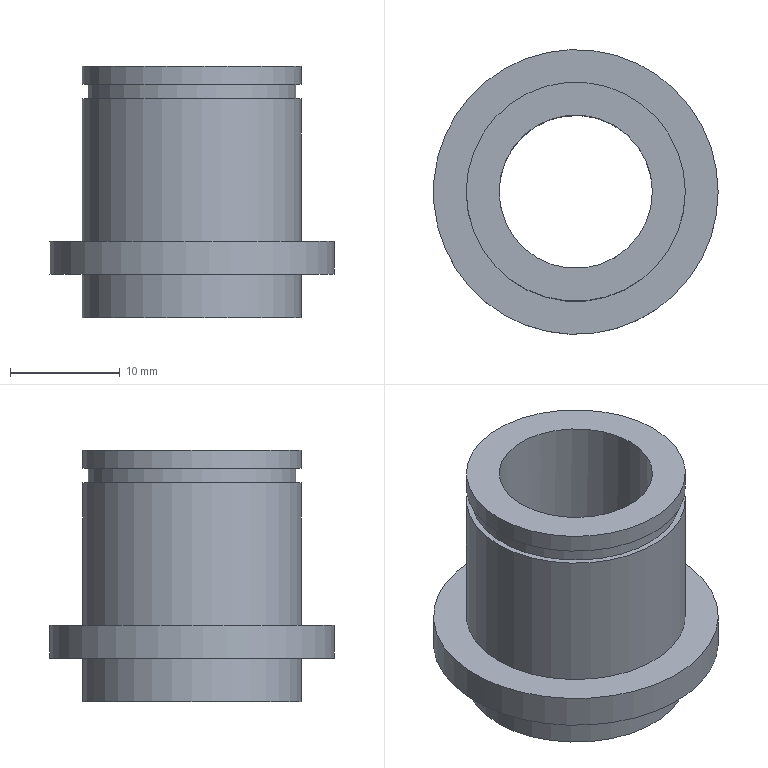Component | NX | 7 | 1 solid | 12 faces | box 26 x 26 x 23 mm | volume 4294 mm3 | plane 6 | cylinder 6 | commonest cylinder face diameters 20 x3 19 x1 26 x1 14 x1
STEP:
#1=CARTESIAN_POINT('',(0.,0.,0.));
#2=DIRECTION('',(0.,0.,1.));
#3=DIRECTION('',(1.,0.,0.));
#4=AXIS2_PLACEMENT_3D('',#1,#2,#3);
#5=CARTESIAN_POINT('',(-11.58,12.798,-36.));
#6=VERTEX_POINT('',#5);
#7=CARTESIAN_POINT('',(2.42,12.798,-36.));
#8=VERTEX_POINT('',#7);
#9=CARTESIAN_POINT('',(-4.58,12.798,-36.));
#10=DIRECTION('',(0.,0.,-1.));
#11=DIRECTION('',(-1.,0.,0.));
#12=AXIS2_PLACEMENT_3D('',#9,#10,#11);
#13=CIRCLE('',#12,7.);
#14=CARTESIAN_POINT('',(-4.58,2.798,-36.));
#15=DIRECTION('',(0.,0.,1.));
#16=DIRECTION('',(-1.,0.,0.));
#17=AXIS2_PLACEMENT_3D('',#14,#15,#16);
#18=PLANE('',#17);
#19=CARTESIAN_POINT('',(7.,-10.));
#20=CARTESIAN_POINT('',(7.,-22.124));
#21=CARTESIAN_POINT('',(-3.5,-16.062));
#22=CARTESIAN_POINT('',(-14.,-10.));
#23=CARTESIAN_POINT('',(-3.5,-3.938));
#24=CARTESIAN_POINT('',(7.,2.124));
#25=CARTESIAN_POINT('',(7.,-10.));
#26=(BOUNDED_CURVE()B_SPLINE_CURVE(2,(#19,#20,#21,#22,#23,#24,#25),.UNSPECIFIED.,.T.,.F.)B_SPLINE_CURVE_WITH_KNOTS((1,2,2,2,2,1),(-2.094,0.,2.094,4.189,6.283,8.378),.UNSPECIFIED.)CURVE()GEOMETRIC_REPRESENTATION_ITEM()RATIONAL_B_SPLINE_CURVE((1.,0.5,1.,0.5,1.,0.5,1.))REPRESENTATION_ITEM(''));
#27=(GEOMETRIC_REPRESENTATION_CONTEXT(2)PARAMETRIC_REPRESENTATION_CONTEXT()REPRESENTATION_CONTEXT('',''));
#28=DEFINITIONAL_REPRESENTATION('',(#26),#27);
#29=PCURVE('',#18,#28);
#30=CARTESIAN_POINT('',(-4.58,12.798,-23.5));
#31=DIRECTION('',(0.,0.,-1.));
#32=DIRECTION('',(1.,0.,0.));
#33=AXIS2_PLACEMENT_3D('',#30,#31,#32);
#34=CYLINDRICAL_SURFACE('',#33,7.);
#35=CARTESIAN_POINT('',(3.142,12.5));
#36=DIRECTION('',(1.,0.));
#37=VECTOR('',#36,1.);
#38=LINE('',#35,#37);
#39=(GEOMETRIC_REPRESENTATION_CONTEXT(2)PARAMETRIC_REPRESENTATION_CONTEXT()REPRESENTATION_CONTEXT('',''));
#40=DEFINITIONAL_REPRESENTATION('',(#38),#39);
#41=PCURVE('',#34,#40);
#42=SURFACE_CURVE('',#13,(#29,#41),.PCURVE_S1.);
#43=EDGE_CURVE('',#6,#8,#42,.T.);
#44=ORIENTED_EDGE('',*,*,#43,.T.);
#45=CARTESIAN_POINT('',(-4.58,12.798,-36.));
#46=DIRECTION('',(0.,0.,-1.));
#47=DIRECTION('',(-1.,0.,0.));
#48=AXIS2_PLACEMENT_3D('',#45,#46,#47);
#49=CIRCLE('',#48,7.);
#50=CARTESIAN_POINT('',(7.,-10.));
#51=CARTESIAN_POINT('',(7.,-22.124));
#52=CARTESIAN_POINT('',(-3.5,-16.062));
#53=CARTESIAN_POINT('',(-14.,-10.));
#54=CARTESIAN_POINT('',(-3.5,-3.938));
#55=CARTESIAN_POINT('',(7.,2.124));
#56=CARTESIAN_POINT('',(7.,-10.));
#57=(BOUNDED_CURVE()B_SPLINE_CURVE(2,(#50,#51,#52,#53,#54,#55,#56),.UNSPECIFIED.,.T.,.F.)B_SPLINE_CURVE_WITH_KNOTS((1,2,2,2,2,1),(-2.094,0.,2.094,4.189,6.283,8.378),.UNSPECIFIED.)CURVE()GEOMETRIC_REPRESENTATION_ITEM()RATIONAL_B_SPLINE_CURVE((1.,0.5,1.,0.5,1.,0.5,1.))REPRESENTATION_ITEM(''));
#58=(GEOMETRIC_REPRESENTATION_CONTEXT(2)PARAMETRIC_REPRESENTATION_CONTEXT()REPRESENTATION_CONTEXT('',''));
#59=DEFINITIONAL_REPRESENTATION('',(#57),#58);
#60=PCURVE('',#18,#59);
#61=CARTESIAN_POINT('',(-3.142,12.5));
#62=DIRECTION('',(1.,0.));
#63=VECTOR('',#62,1.);
#64=LINE('',#61,#63);
#65=(GEOMETRIC_REPRESENTATION_CONTEXT(2)PARAMETRIC_REPRESENTATION_CONTEXT()REPRESENTATION_CONTEXT('',''));
#66=DEFINITIONAL_REPRESENTATION('',(#64),#65);
#67=PCURVE('',#34,#66);
#68=SURFACE_CURVE('',#49,(#60,#67),.PCURVE_S1.);
#69=EDGE_CURVE('',#8,#6,#68,.T.);
#70=ORIENTED_EDGE('',*,*,#69,.T.);
#71=EDGE_LOOP('',(#44,#70));
#72=FACE_BOUND('',#71,.T.);
#73=CARTESIAN_POINT('',(5.42,12.798,-36.));
#74=VERTEX_POINT('',#73);
#75=CARTESIAN_POINT('',(-4.58,12.798,-36.));
#76=DIRECTION('',(0.,0.,-1.));
#77=DIRECTION('',(1.,0.,0.));
#78=AXIS2_PLACEMENT_3D('',#75,#76,#77);
#79=CIRCLE('',#78,10.);
#80=CARTESIAN_POINT('',(-10.,-10.));
#81=CARTESIAN_POINT('',(-10.,7.321));
#82=CARTESIAN_POINT('',(5.,-1.34));
#83=CARTESIAN_POINT('',(20.,-10.));
#84=CARTESIAN_POINT('',(5.,-18.66));
#85=CARTESIAN_POINT('',(-10.,-27.321));
#86=CARTESIAN_POINT('',(-10.,-10.));
#87=(BOUNDED_CURVE()B_SPLINE_CURVE(2,(#80,#81,#82,#83,#84,#85,#86),.UNSPECIFIED.,.T.,.F.)B_SPLINE_CURVE_WITH_KNOTS((1,2,2,2,2,1),(-2.094,0.,2.094,4.189,6.283,8.378),.UNSPECIFIED.)CURVE()GEOMETRIC_REPRESENTATION_ITEM()RATIONAL_B_SPLINE_CURVE((1.,0.5,1.,0.5,1.,0.5,1.))REPRESENTATION_ITEM(''));
#88=(GEOMETRIC_REPRESENTATION_CONTEXT(2)PARAMETRIC_REPRESENTATION_CONTEXT()REPRESENTATION_CONTEXT('',''));
#89=DEFINITIONAL_REPRESENTATION('',(#87),#88);
#90=PCURVE('',#18,#89);
#91=CARTESIAN_POINT('',(-4.58,12.798,-36.));
#92=DIRECTION('',(0.,0.,-1.));
#93=DIRECTION('',(1.,0.,0.));
#94=AXIS2_PLACEMENT_3D('',#91,#92,#93);
#95=CYLINDRICAL_SURFACE('',#94,10.);
#96=CARTESIAN_POINT('',(0.,0.));
#97=DIRECTION('',(1.,0.));
#98=VECTOR('',#97,1.);
#99=LINE('',#96,#98);
#100=(GEOMETRIC_REPRESENTATION_CONTEXT(2)PARAMETRIC_REPRESENTATION_CONTEXT()REPRESENTATION_CONTEXT('',''));
#101=DEFINITIONAL_REPRESENTATION('',(#99),#100);
#102=PCURVE('',#95,#101);
#103=SURFACE_CURVE('',#79,(#90,#102),.PCURVE_S1.);
#104=EDGE_CURVE('',#74,#74,#103,.T.);
#105=ORIENTED_EDGE('',*,*,#104,.F.);
#106=EDGE_LOOP('',(#105));
#107=FACE_BOUND('',#106,.T.);
#108=ADVANCED_FACE('',(#72,#107),#18,.T.);
#109=ORIENTED_EDGE('',*,*,#104,.T.);
#110=CARTESIAN_POINT('',(5.42,12.798,-37.65));
#111=VERTEX_POINT('',#110);
#112=CARTESIAN_POINT('',(5.42,12.798,-36.));
#113=CARTESIAN_POINT('',(5.42,12.798,-37.65));
#114=B_SPLINE_CURVE_WITH_KNOTS('',1,(#112,#113),.UNSPECIFIED.,.F.,.F.,(2,2),(0.,1.65),.PIECEWISE_BEZIER_KNOTS.);
#115=CARTESIAN_POINT('',(6.283,0.));
#116=DIRECTION('',(0.,1.));
#117=VECTOR('',#116,1.);
#118=LINE('',#115,#117);
#119=(GEOMETRIC_REPRESENTATION_CONTEXT(2)PARAMETRIC_REPRESENTATION_CONTEXT()REPRESENTATION_CONTEXT('',''));
#120=DEFINITIONAL_REPRESENTATION('',(#118),#119);
#121=PCURVE('',#95,#120);
#122=CARTESIAN_POINT('',(0.,0.));
#123=DIRECTION('',(0.,1.));
#124=VECTOR('',#123,1.);
#125=LINE('',#122,#124);
#126=(GEOMETRIC_REPRESENTATION_CONTEXT(2)PARAMETRIC_REPRESENTATION_CONTEXT()REPRESENTATION_CONTEXT('',''));
#127=DEFINITIONAL_REPRESENTATION('',(#125),#126);
#128=PCURVE('',#95,#127);
#129=SEAM_CURVE('',#114,(#121,#128),.PCURVE_S1.);
#130=EDGE_CURVE('',#74,#111,#129,.T.);
#131=ORIENTED_EDGE('',*,*,#130,.T.);
#132=CARTESIAN_POINT('',(-4.58,12.798,-37.65));
#133=DIRECTION('',(0.,0.,-1.));
#134=DIRECTION('',(1.,0.,0.));
#135=AXIS2_PLACEMENT_3D('',#132,#133,#134);
#136=CIRCLE('',#135,10.);
#137=CARTESIAN_POINT('',(0.,1.65));
#138=DIRECTION('',(1.,0.));
#139=VECTOR('',#138,1.);
#140=LINE('',#137,#139);
#141=(GEOMETRIC_REPRESENTATION_CONTEXT(2)PARAMETRIC_REPRESENTATION_CONTEXT()REPRESENTATION_CONTEXT('',''));
#142=DEFINITIONAL_REPRESENTATION('',(#140),#141);
#143=PCURVE('',#95,#142);
#144=CARTESIAN_POINT('',(-4.58,3.298,-37.65));
#145=DIRECTION('',(0.,0.,-1.));
#146=DIRECTION('',(1.,0.,0.));
#147=AXIS2_PLACEMENT_3D('',#144,#145,#146);
#148=PLANE('',#147);
#149=CARTESIAN_POINT('',(0.,-9.5));
#150=DIRECTION('',(1.,0.));
#151=AXIS2_PLACEMENT_2D('',#149,#150);
#152=CIRCLE('',#151,10.);
#153=(GEOMETRIC_REPRESENTATION_CONTEXT(2)PARAMETRIC_REPRESENTATION_CONTEXT()REPRESENTATION_CONTEXT('',''));
#154=DEFINITIONAL_REPRESENTATION('',(#152),#153);
#155=PCURVE('',#148,#154);
#156=SURFACE_CURVE('',#136,(#143,#155),.PCURVE_S1.);
#157=EDGE_CURVE('',#111,#111,#156,.T.);
#158=ORIENTED_EDGE('',*,*,#157,.F.);
#159=ORIENTED_EDGE('',*,*,#130,.F.);
#160=EDGE_LOOP('',(#109,#131,#158,#159));
#161=FACE_BOUND('',#160,.T.);
#162=ADVANCED_FACE('',(#161),#95,.T.);
#163=ORIENTED_EDGE('',*,*,#157,.T.);
#164=EDGE_LOOP('',(#163));
#165=FACE_BOUND('',#164,.T.);
#166=CARTESIAN_POINT('',(4.92,12.798,-37.65));
#167=VERTEX_POINT('',#166);
#168=CARTESIAN_POINT('',(-4.58,12.798,-37.65));
#169=DIRECTION('',(0.,0.,-1.));
#170=DIRECTION('',(1.,0.,0.));
#171=AXIS2_PLACEMENT_3D('',#168,#169,#170);
#172=CIRCLE('',#171,9.5);
#173=CARTESIAN_POINT('',(0.,-9.5));
#174=DIRECTION('',(1.,0.));
#175=AXIS2_PLACEMENT_2D('',#173,#174);
#176=CIRCLE('',#175,9.5);
#177=(GEOMETRIC_REPRESENTATION_CONTEXT(2)PARAMETRIC_REPRESENTATION_CONTEXT()REPRESENTATION_CONTEXT('',''));
#178=DEFINITIONAL_REPRESENTATION('',(#176),#177);
#179=PCURVE('',#148,#178);
#180=CARTESIAN_POINT('',(-4.58,12.798,-36.));
#181=DIRECTION('',(0.,0.,-1.));
#182=DIRECTION('',(1.,0.,0.));
#183=AXIS2_PLACEMENT_3D('',#180,#181,#182);
#184=CYLINDRICAL_SURFACE('',#183,9.5);
#185=CARTESIAN_POINT('',(0.,1.65));
#186=DIRECTION('',(1.,0.));
#187=VECTOR('',#186,1.);
#188=LINE('',#185,#187);
#189=(GEOMETRIC_REPRESENTATION_CONTEXT(2)PARAMETRIC_REPRESENTATION_CONTEXT()REPRESENTATION_CONTEXT('',''));
#190=DEFINITIONAL_REPRESENTATION('',(#188),#189);
#191=PCURVE('',#184,#190);
#192=SURFACE_CURVE('',#172,(#179,#191),.PCURVE_S1.);
#193=EDGE_CURVE('',#167,#167,#192,.T.);
#194=ORIENTED_EDGE('',*,*,#193,.F.);
#195=EDGE_LOOP('',(#194));
#196=FACE_BOUND('',#195,.T.);
#197=ADVANCED_FACE('',(#165,#196),#148,.T.);
#198=ORIENTED_EDGE('',*,*,#193,.T.);
#199=CARTESIAN_POINT('',(4.92,12.798,-39.));
#200=VERTEX_POINT('',#199);
#201=CARTESIAN_POINT('',(4.92,12.798,-37.65));
#202=CARTESIAN_POINT('',(4.92,12.798,-39.));
#203=B_SPLINE_CURVE_WITH_KNOTS('',1,(#201,#202),.UNSPECIFIED.,.F.,.F.,(2,2),(1.65,3.),.PIECEWISE_BEZIER_KNOTS.);
#204=CARTESIAN_POINT('',(6.283,0.));
#205=DIRECTION('',(0.,1.));
#206=VECTOR('',#205,1.);
#207=LINE('',#204,#206);
#208=(GEOMETRIC_REPRESENTATION_CONTEXT(2)PARAMETRIC_REPRESENTATION_CONTEXT()REPRESENTATION_CONTEXT('',''));
#209=DEFINITIONAL_REPRESENTATION('',(#207),#208);
#210=PCURVE('',#184,#209);
#211=CARTESIAN_POINT('',(0.,0.));
#212=DIRECTION('',(0.,1.));
#213=VECTOR('',#212,1.);
#214=LINE('',#211,#213);
#215=(GEOMETRIC_REPRESENTATION_CONTEXT(2)PARAMETRIC_REPRESENTATION_CONTEXT()REPRESENTATION_CONTEXT('',''));
#216=DEFINITIONAL_REPRESENTATION('',(#214),#215);
#217=PCURVE('',#184,#216);
#218=SEAM_CURVE('',#203,(#210,#217),.PCURVE_S1.);
#219=EDGE_CURVE('',#167,#200,#218,.T.);
#220=ORIENTED_EDGE('',*,*,#219,.T.);
#221=CARTESIAN_POINT('',(-4.58,12.798,-39.));
#222=DIRECTION('',(0.,0.,-1.));
#223=DIRECTION('',(1.,0.,0.));
#224=AXIS2_PLACEMENT_3D('',#221,#222,#223);
#225=CIRCLE('',#224,9.5);
#226=CARTESIAN_POINT('',(0.,3.));
#227=DIRECTION('',(1.,0.));
#228=VECTOR('',#227,1.);
#229=LINE('',#226,#228);
#230=(GEOMETRIC_REPRESENTATION_CONTEXT(2)PARAMETRIC_REPRESENTATION_CONTEXT()REPRESENTATION_CONTEXT('',''));
#231=DEFINITIONAL_REPRESENTATION('',(#229),#230);
#232=PCURVE('',#184,#231);
#233=CARTESIAN_POINT('',(-4.58,2.798,-39.));
#234=DIRECTION('',(0.,0.,1.));
#235=DIRECTION('',(-1.,0.,0.));
#236=AXIS2_PLACEMENT_3D('',#233,#234,#235);
#237=PLANE('',#236);
#238=CARTESIAN_POINT('',(-9.5,-10.));
#239=CARTESIAN_POINT('',(-9.5,6.454));
#240=CARTESIAN_POINT('',(4.75,-1.773));
#241=CARTESIAN_POINT('',(19.,-10.));
#242=CARTESIAN_POINT('',(4.75,-18.227));
#243=CARTESIAN_POINT('',(-9.5,-26.454));
#244=CARTESIAN_POINT('',(-9.5,-10.));
#245=(BOUNDED_CURVE()B_SPLINE_CURVE(2,(#238,#239,#240,#241,#242,#243,#244),.UNSPECIFIED.,.T.,.F.)B_SPLINE_CURVE_WITH_KNOTS((1,2,2,2,2,1),(-2.094,0.,2.094,4.189,6.283,8.378),.UNSPECIFIED.)CURVE()GEOMETRIC_REPRESENTATION_ITEM()RATIONAL_B_SPLINE_CURVE((1.,0.5,1.,0.5,1.,0.5,1.))REPRESENTATION_ITEM(''));
#246=(GEOMETRIC_REPRESENTATION_CONTEXT(2)PARAMETRIC_REPRESENTATION_CONTEXT()REPRESENTATION_CONTEXT('',''));
#247=DEFINITIONAL_REPRESENTATION('',(#245),#246);
#248=PCURVE('',#237,#247);
#249=SURFACE_CURVE('',#225,(#232,#248),.PCURVE_S1.);
#250=EDGE_CURVE('',#200,#200,#249,.T.);
#251=ORIENTED_EDGE('',*,*,#250,.F.);
#252=ORIENTED_EDGE('',*,*,#219,.F.);
#253=EDGE_LOOP('',(#198,#220,#251,#252));
#254=FACE_BOUND('',#253,.T.);
#255=ADVANCED_FACE('',(#254),#184,.T.);
#256=ORIENTED_EDGE('',*,*,#250,.T.);
#257=EDGE_LOOP('',(#256));
#258=FACE_BOUND('',#257,.T.);
#259=CARTESIAN_POINT('',(5.42,12.798,-39.));
#260=VERTEX_POINT('',#259);
#261=CARTESIAN_POINT('',(-4.58,12.798,-39.));
#262=DIRECTION('',(0.,0.,-1.));
#263=DIRECTION('',(1.,0.,0.));
#264=AXIS2_PLACEMENT_3D('',#261,#262,#263);
#265=CIRCLE('',#264,10.);
#266=CARTESIAN_POINT('',(-10.,-10.));
#267=CARTESIAN_POINT('',(-10.,7.321));
#268=CARTESIAN_POINT('',(5.,-1.34));
#269=CARTESIAN_POINT('',(20.,-10.));
#270=CARTESIAN_POINT('',(5.,-18.66));
#271=CARTESIAN_POINT('',(-10.,-27.321));
#272=CARTESIAN_POINT('',(-10.,-10.));
#273=(BOUNDED_CURVE()B_SPLINE_CURVE(2,(#266,#267,#268,#269,#270,#271,#272),.UNSPECIFIED.,.T.,.F.)B_SPLINE_CURVE_WITH_KNOTS((1,2,2,2,2,1),(-2.094,0.,2.094,4.189,6.283,8.378),.UNSPECIFIED.)CURVE()GEOMETRIC_REPRESENTATION_ITEM()RATIONAL_B_SPLINE_CURVE((1.,0.5,1.,0.5,1.,0.5,1.))REPRESENTATION_ITEM(''));
#274=(GEOMETRIC_REPRESENTATION_CONTEXT(2)PARAMETRIC_REPRESENTATION_CONTEXT()REPRESENTATION_CONTEXT('',''));
#275=DEFINITIONAL_REPRESENTATION('',(#273),#274);
#276=PCURVE('',#237,#275);
#277=CARTESIAN_POINT('',(-4.58,12.798,-36.));
#278=DIRECTION('',(0.,0.,-1.));
#279=DIRECTION('',(1.,0.,0.));
#280=AXIS2_PLACEMENT_3D('',#277,#278,#279);
#281=CYLINDRICAL_SURFACE('',#280,10.);
#282=CARTESIAN_POINT('',(0.,3.));
#283=DIRECTION('',(1.,0.));
#284=VECTOR('',#283,1.);
#285=LINE('',#282,#284);
#286=(GEOMETRIC_REPRESENTATION_CONTEXT(2)PARAMETRIC_REPRESENTATION_CONTEXT()REPRESENTATION_CONTEXT('',''));
#287=DEFINITIONAL_REPRESENTATION('',(#285),#286);
#288=PCURVE('',#281,#287);
#289=SURFACE_CURVE('',#265,(#276,#288),.PCURVE_S1.);
#290=EDGE_CURVE('',#260,#260,#289,.T.);
#291=ORIENTED_EDGE('',*,*,#290,.F.);
#292=EDGE_LOOP('',(#291));
#293=FACE_BOUND('',#292,.T.);
#294=ADVANCED_FACE('',(#258,#293),#237,.T.);
#295=ORIENTED_EDGE('',*,*,#290,.T.);
#296=CARTESIAN_POINT('',(5.42,12.798,-52.));
#297=VERTEX_POINT('',#296);
#298=CARTESIAN_POINT('',(5.42,12.798,-39.));
#299=CARTESIAN_POINT('',(5.42,12.798,-52.));
#300=B_SPLINE_CURVE_WITH_KNOTS('',1,(#298,#299),.UNSPECIFIED.,.F.,.F.,(2,2),(3.,16.),.PIECEWISE_BEZIER_KNOTS.);
#301=CARTESIAN_POINT('',(6.283,0.));
#302=DIRECTION('',(0.,1.));
#303=VECTOR('',#302,1.);
#304=LINE('',#301,#303);
#305=(GEOMETRIC_REPRESENTATION_CONTEXT(2)PARAMETRIC_REPRESENTATION_CONTEXT()REPRESENTATION_CONTEXT('',''));
#306=DEFINITIONAL_REPRESENTATION('',(#304),#305);
#307=PCURVE('',#281,#306);
#308=CARTESIAN_POINT('',(0.,0.));
#309=DIRECTION('',(0.,1.));
#310=VECTOR('',#309,1.);
#311=LINE('',#308,#310);
#312=(GEOMETRIC_REPRESENTATION_CONTEXT(2)PARAMETRIC_REPRESENTATION_CONTEXT()REPRESENTATION_CONTEXT('',''));
#313=DEFINITIONAL_REPRESENTATION('',(#311),#312);
#314=PCURVE('',#281,#313);
#315=SEAM_CURVE('',#300,(#307,#314),.PCURVE_S1.);
#316=EDGE_CURVE('',#260,#297,#315,.T.);
#317=ORIENTED_EDGE('',*,*,#316,.T.);
#318=CARTESIAN_POINT('',(-4.58,12.798,-52.));
#319=DIRECTION('',(0.,0.,-1.));
#320=DIRECTION('',(1.,0.,0.));
#321=AXIS2_PLACEMENT_3D('',#318,#319,#320);
#322=CIRCLE('',#321,10.);
#323=CARTESIAN_POINT('',(0.,16.));
#324=DIRECTION('',(1.,0.));
#325=VECTOR('',#324,1.);
#326=LINE('',#323,#325);
#327=(GEOMETRIC_REPRESENTATION_CONTEXT(2)PARAMETRIC_REPRESENTATION_CONTEXT()REPRESENTATION_CONTEXT('',''));
#328=DEFINITIONAL_REPRESENTATION('',(#326),#327);
#329=PCURVE('',#281,#328);
#330=CARTESIAN_POINT('',(-4.58,-0.2019,-52.));
#331=DIRECTION('',(0.,0.,1.));
#332=DIRECTION('',(-1.,0.,0.));
#333=AXIS2_PLACEMENT_3D('',#330,#331,#332);
#334=PLANE('',#333);
#335=CARTESIAN_POINT('',(-10.,-13.));
#336=CARTESIAN_POINT('',(-10.,4.321));
#337=CARTESIAN_POINT('',(5.,-4.34));
#338=CARTESIAN_POINT('',(20.,-13.));
#339=CARTESIAN_POINT('',(5.,-21.66));
#340=CARTESIAN_POINT('',(-10.,-30.321));
#341=CARTESIAN_POINT('',(-10.,-13.));
#342=(BOUNDED_CURVE()B_SPLINE_CURVE(2,(#335,#336,#337,#338,#339,#340,#341),.UNSPECIFIED.,.T.,.F.)B_SPLINE_CURVE_WITH_KNOTS((1,2,2,2,2,1),(-2.094,0.,2.094,4.189,6.283,8.378),.UNSPECIFIED.)CURVE()GEOMETRIC_REPRESENTATION_ITEM()RATIONAL_B_SPLINE_CURVE((1.,0.5,1.,0.5,1.,0.5,1.))REPRESENTATION_ITEM(''));
#343=(GEOMETRIC_REPRESENTATION_CONTEXT(2)PARAMETRIC_REPRESENTATION_CONTEXT()REPRESENTATION_CONTEXT('',''));
#344=DEFINITIONAL_REPRESENTATION('',(#342),#343);
#345=PCURVE('',#334,#344);
#346=SURFACE_CURVE('',#322,(#329,#345),.PCURVE_S1.);
#347=EDGE_CURVE('',#297,#297,#346,.T.);
#348=ORIENTED_EDGE('',*,*,#347,.F.);
#349=ORIENTED_EDGE('',*,*,#316,.F.);
#350=EDGE_LOOP('',(#295,#317,#348,#349));
#351=FACE_BOUND('',#350,.T.);
#352=ADVANCED_FACE('',(#351),#281,.T.);
#353=ORIENTED_EDGE('',*,*,#347,.T.);
#354=EDGE_LOOP('',(#353));
#355=FACE_BOUND('',#354,.T.);
#356=CARTESIAN_POINT('',(8.42,12.798,-52.));
#357=VERTEX_POINT('',#356);
#358=CARTESIAN_POINT('',(-4.58,12.798,-52.));
#359=DIRECTION('',(0.,0.,-1.));
#360=DIRECTION('',(1.,0.,0.));
#361=AXIS2_PLACEMENT_3D('',#358,#359,#360);
#362=CIRCLE('',#361,13.);
#363=CARTESIAN_POINT('',(-13.,-13.));
#364=CARTESIAN_POINT('',(-13.,9.517));
#365=CARTESIAN_POINT('',(6.5,-1.742));
#366=CARTESIAN_POINT('',(26.,-13.));
#367=CARTESIAN_POINT('',(6.5,-24.258));
#368=CARTESIAN_POINT('',(-13.,-35.517));
#369=CARTESIAN_POINT('',(-13.,-13.));
#370=(BOUNDED_CURVE()B_SPLINE_CURVE(2,(#363,#364,#365,#366,#367,#368,#369),.UNSPECIFIED.,.T.,.F.)B_SPLINE_CURVE_WITH_KNOTS((1,2,2,2,2,1),(-2.094,0.,2.094,4.189,6.283,8.378),.UNSPECIFIED.)CURVE()GEOMETRIC_REPRESENTATION_ITEM()RATIONAL_B_SPLINE_CURVE((1.,0.5,1.,0.5,1.,0.5,1.))REPRESENTATION_ITEM(''));
#371=(GEOMETRIC_REPRESENTATION_CONTEXT(2)PARAMETRIC_REPRESENTATION_CONTEXT()REPRESENTATION_CONTEXT('',''));
#372=DEFINITIONAL_REPRESENTATION('',(#370),#371);
#373=PCURVE('',#334,#372);
#374=CARTESIAN_POINT('',(-4.58,12.798,-36.));
#375=DIRECTION('',(0.,0.,-1.));
#376=DIRECTION('',(1.,0.,0.));
#377=AXIS2_PLACEMENT_3D('',#374,#375,#376);
#378=CYLINDRICAL_SURFACE('',#377,13.);
#379=CARTESIAN_POINT('',(0.,16.));
#380=DIRECTION('',(1.,0.));
#381=VECTOR('',#380,1.);
#382=LINE('',#379,#381);
#383=(GEOMETRIC_REPRESENTATION_CONTEXT(2)PARAMETRIC_REPRESENTATION_CONTEXT()REPRESENTATION_CONTEXT('',''));
#384=DEFINITIONAL_REPRESENTATION('',(#382),#383);
#385=PCURVE('',#378,#384);
#386=SURFACE_CURVE('',#362,(#373,#385),.PCURVE_S1.);
#387=EDGE_CURVE('',#357,#357,#386,.T.);
#388=ORIENTED_EDGE('',*,*,#387,.F.);
#389=EDGE_LOOP('',(#388));
#390=FACE_BOUND('',#389,.T.);
#391=ADVANCED_FACE('',(#355,#390),#334,.T.);
#392=ORIENTED_EDGE('',*,*,#387,.T.);
#393=CARTESIAN_POINT('',(8.42,12.798,-55.));
#394=VERTEX_POINT('',#393);
#395=CARTESIAN_POINT('',(8.42,12.798,-52.));
#396=CARTESIAN_POINT('',(8.42,12.798,-55.));
#397=B_SPLINE_CURVE_WITH_KNOTS('',1,(#395,#396),.UNSPECIFIED.,.F.,.F.,(2,2),(16.,19.),.PIECEWISE_BEZIER_KNOTS.);
#398=CARTESIAN_POINT('',(6.283,0.));
#399=DIRECTION('',(0.,1.));
#400=VECTOR('',#399,1.);
#401=LINE('',#398,#400);
#402=(GEOMETRIC_REPRESENTATION_CONTEXT(2)PARAMETRIC_REPRESENTATION_CONTEXT()REPRESENTATION_CONTEXT('',''));
#403=DEFINITIONAL_REPRESENTATION('',(#401),#402);
#404=PCURVE('',#378,#403);
#405=CARTESIAN_POINT('',(0.,0.));
#406=DIRECTION('',(0.,1.));
#407=VECTOR('',#406,1.);
#408=LINE('',#405,#407);
#409=(GEOMETRIC_REPRESENTATION_CONTEXT(2)PARAMETRIC_REPRESENTATION_CONTEXT()REPRESENTATION_CONTEXT('',''));
#410=DEFINITIONAL_REPRESENTATION('',(#408),#409);
#411=PCURVE('',#378,#410);
#412=SEAM_CURVE('',#397,(#404,#411),.PCURVE_S1.);
#413=EDGE_CURVE('',#357,#394,#412,.T.);
#414=ORIENTED_EDGE('',*,*,#413,.T.);
#415=CARTESIAN_POINT('',(-4.58,12.798,-55.));
#416=DIRECTION('',(0.,0.,-1.));
#417=DIRECTION('',(1.,0.,0.));
#418=AXIS2_PLACEMENT_3D('',#415,#416,#417);
#419=CIRCLE('',#418,13.);
#420=CARTESIAN_POINT('',(0.,19.));
#421=DIRECTION('',(1.,0.));
#422=VECTOR('',#421,1.);
#423=LINE('',#420,#422);
#424=(GEOMETRIC_REPRESENTATION_CONTEXT(2)PARAMETRIC_REPRESENTATION_CONTEXT()REPRESENTATION_CONTEXT('',''));
#425=DEFINITIONAL_REPRESENTATION('',(#423),#424);
#426=PCURVE('',#378,#425);
#427=CARTESIAN_POINT('',(-4.58,2.798,-55.));
#428=DIRECTION('',(0.,0.,-1.));
#429=DIRECTION('',(1.,0.,0.));
#430=AXIS2_PLACEMENT_3D('',#427,#428,#429);
#431=PLANE('',#430);
#432=CARTESIAN_POINT('',(0.,-10.));
#433=DIRECTION('',(1.,0.));
#434=AXIS2_PLACEMENT_2D('',#432,#433);
#435=CIRCLE('',#434,13.);
#436=(GEOMETRIC_REPRESENTATION_CONTEXT(2)PARAMETRIC_REPRESENTATION_CONTEXT()REPRESENTATION_CONTEXT('',''));
#437=DEFINITIONAL_REPRESENTATION('',(#435),#436);
#438=PCURVE('',#431,#437);
#439=SURFACE_CURVE('',#419,(#426,#438),.PCURVE_S1.);
#440=EDGE_CURVE('',#394,#394,#439,.T.);
#441=ORIENTED_EDGE('',*,*,#440,.F.);
#442=ORIENTED_EDGE('',*,*,#413,.F.);
#443=EDGE_LOOP('',(#392,#414,#441,#442));
#444=FACE_BOUND('',#443,.T.);
#445=ADVANCED_FACE('',(#444),#378,.T.);
#446=ORIENTED_EDGE('',*,*,#440,.T.);
#447=EDGE_LOOP('',(#446));
#448=FACE_BOUND('',#447,.T.);
#449=CARTESIAN_POINT('',(5.42,12.798,-55.));
#450=VERTEX_POINT('',#449);
#451=CARTESIAN_POINT('',(-4.58,12.798,-55.));
#452=DIRECTION('',(0.,0.,-1.));
#453=DIRECTION('',(1.,0.,0.));
#454=AXIS2_PLACEMENT_3D('',#451,#452,#453);
#455=CIRCLE('',#454,10.);
#456=CARTESIAN_POINT('',(0.,-10.));
#457=DIRECTION('',(1.,0.));
#458=AXIS2_PLACEMENT_2D('',#456,#457);
#459=CIRCLE('',#458,10.);
#460=(GEOMETRIC_REPRESENTATION_CONTEXT(2)PARAMETRIC_REPRESENTATION_CONTEXT()REPRESENTATION_CONTEXT('',''));
#461=DEFINITIONAL_REPRESENTATION('',(#459),#460);
#462=PCURVE('',#431,#461);
#463=CARTESIAN_POINT('',(-4.58,12.798,-36.));
#464=DIRECTION('',(0.,0.,-1.));
#465=DIRECTION('',(1.,0.,0.));
#466=AXIS2_PLACEMENT_3D('',#463,#464,#465);
#467=CYLINDRICAL_SURFACE('',#466,10.);
#468=CARTESIAN_POINT('',(0.,19.));
#469=DIRECTION('',(1.,0.));
#470=VECTOR('',#469,1.);
#471=LINE('',#468,#470);
#472=(GEOMETRIC_REPRESENTATION_CONTEXT(2)PARAMETRIC_REPRESENTATION_CONTEXT()REPRESENTATION_CONTEXT('',''));
#473=DEFINITIONAL_REPRESENTATION('',(#471),#472);
#474=PCURVE('',#467,#473);
#475=SURFACE_CURVE('',#455,(#462,#474),.PCURVE_S1.);
#476=EDGE_CURVE('',#450,#450,#475,.T.);
#477=ORIENTED_EDGE('',*,*,#476,.F.);
#478=EDGE_LOOP('',(#477));
#479=FACE_BOUND('',#478,.T.);
#480=ADVANCED_FACE('',(#448,#479),#431,.T.);
#481=ORIENTED_EDGE('',*,*,#476,.T.);
#482=CARTESIAN_POINT('',(5.42,12.798,-59.));
#483=VERTEX_POINT('',#482);
#484=CARTESIAN_POINT('',(5.42,12.798,-55.));
#485=CARTESIAN_POINT('',(5.42,12.798,-59.));
#486=B_SPLINE_CURVE_WITH_KNOTS('',1,(#484,#485),.UNSPECIFIED.,.F.,.F.,(2,2),(19.,23.),.PIECEWISE_BEZIER_KNOTS.);
#487=CARTESIAN_POINT('',(6.283,0.));
#488=DIRECTION('',(0.,1.));
#489=VECTOR('',#488,1.);
#490=LINE('',#487,#489);
#491=(GEOMETRIC_REPRESENTATION_CONTEXT(2)PARAMETRIC_REPRESENTATION_CONTEXT()REPRESENTATION_CONTEXT('',''));
#492=DEFINITIONAL_REPRESENTATION('',(#490),#491);
#493=PCURVE('',#467,#492);
#494=CARTESIAN_POINT('',(0.,0.));
#495=DIRECTION('',(0.,1.));
#496=VECTOR('',#495,1.);
#497=LINE('',#494,#496);
#498=(GEOMETRIC_REPRESENTATION_CONTEXT(2)PARAMETRIC_REPRESENTATION_CONTEXT()REPRESENTATION_CONTEXT('',''));
#499=DEFINITIONAL_REPRESENTATION('',(#497),#498);
#500=PCURVE('',#467,#499);
#501=SEAM_CURVE('',#486,(#493,#500),.PCURVE_S1.);
#502=EDGE_CURVE('',#450,#483,#501,.T.);
#503=ORIENTED_EDGE('',*,*,#502,.T.);
#504=CARTESIAN_POINT('',(-4.58,12.798,-59.));
#505=DIRECTION('',(0.,0.,-1.));
#506=DIRECTION('',(1.,0.,0.));
#507=AXIS2_PLACEMENT_3D('',#504,#505,#506);
#508=CIRCLE('',#507,10.);
#509=CARTESIAN_POINT('',(0.,23.));
#510=DIRECTION('',(1.,0.));
#511=VECTOR('',#510,1.);
#512=LINE('',#509,#511);
#513=(GEOMETRIC_REPRESENTATION_CONTEXT(2)PARAMETRIC_REPRESENTATION_CONTEXT()REPRESENTATION_CONTEXT('',''));
#514=DEFINITIONAL_REPRESENTATION('',(#512),#513);
#515=PCURVE('',#467,#514);
#516=CARTESIAN_POINT('',(-4.58,12.798,-59.));
#517=DIRECTION('',(0.,0.,-1.));
#518=DIRECTION('',(1.,0.,0.));
#519=AXIS2_PLACEMENT_3D('',#516,#517,#518);
#520=PLANE('',#519);
#521=CARTESIAN_POINT('',(0.,0.));
#522=DIRECTION('',(1.,0.));
#523=AXIS2_PLACEMENT_2D('',#521,#522);
#524=CIRCLE('',#523,10.);
#525=(GEOMETRIC_REPRESENTATION_CONTEXT(2)PARAMETRIC_REPRESENTATION_CONTEXT()REPRESENTATION_CONTEXT('',''));
#526=DEFINITIONAL_REPRESENTATION('',(#524),#525);
#527=PCURVE('',#520,#526);
#528=SURFACE_CURVE('',#508,(#515,#527),.PCURVE_S1.);
#529=EDGE_CURVE('',#483,#483,#528,.T.);
#530=ORIENTED_EDGE('',*,*,#529,.F.);
#531=ORIENTED_EDGE('',*,*,#502,.F.);
#532=EDGE_LOOP('',(#481,#503,#530,#531));
#533=FACE_BOUND('',#532,.T.);
#534=ADVANCED_FACE('',(#533),#467,.T.);
#535=CARTESIAN_POINT('',(2.42,12.798,-59.));
#536=VERTEX_POINT('',#535);
#537=CARTESIAN_POINT('',(-4.58,12.798,-59.));
#538=DIRECTION('',(0.,0.,1.));
#539=DIRECTION('',(1.,0.,0.));
#540=AXIS2_PLACEMENT_3D('',#537,#538,#539);
#541=CIRCLE('',#540,7.);
#542=CARTESIAN_POINT('',(7.,0.));
#543=CARTESIAN_POINT('',(7.,-12.124));
#544=CARTESIAN_POINT('',(-3.5,-6.062));
#545=CARTESIAN_POINT('',(-14.,-0.));
#546=CARTESIAN_POINT('',(-3.5,6.062));
#547=CARTESIAN_POINT('',(7.,12.124));
#548=CARTESIAN_POINT('',(7.,0.));
#549=(BOUNDED_CURVE()B_SPLINE_CURVE(2,(#542,#543,#544,#545,#546,#547,#548),.UNSPECIFIED.,.T.,.F.)B_SPLINE_CURVE_WITH_KNOTS((1,2,2,2,2,1),(-2.094,0.,2.094,4.189,6.283,8.378),.UNSPECIFIED.)CURVE()GEOMETRIC_REPRESENTATION_ITEM()RATIONAL_B_SPLINE_CURVE((1.,0.5,1.,0.5,1.,0.5,1.))REPRESENTATION_ITEM(''));
#550=(GEOMETRIC_REPRESENTATION_CONTEXT(2)PARAMETRIC_REPRESENTATION_CONTEXT()REPRESENTATION_CONTEXT('',''));
#551=DEFINITIONAL_REPRESENTATION('',(#549),#550);
#552=PCURVE('',#520,#551);
#553=CARTESIAN_POINT('',(6.283,35.5));
#554=DIRECTION('',(-1.,0.));
#555=VECTOR('',#554,1.);
#556=LINE('',#553,#555);
#557=(GEOMETRIC_REPRESENTATION_CONTEXT(2)PARAMETRIC_REPRESENTATION_CONTEXT()REPRESENTATION_CONTEXT('',''));
#558=DEFINITIONAL_REPRESENTATION('',(#556),#557);
#559=PCURVE('',#34,#558);
#560=SURFACE_CURVE('',#541,(#552,#559),.PCURVE_S1.);
#561=EDGE_CURVE('',#536,#536,#560,.T.);
#562=ORIENTED_EDGE('',*,*,#561,.T.);
#563=EDGE_LOOP('',(#562));
#564=FACE_BOUND('',#563,.T.);
#565=ORIENTED_EDGE('',*,*,#529,.T.);
#566=EDGE_LOOP('',(#565));
#567=FACE_BOUND('',#566,.T.);
#568=ADVANCED_FACE('',(#564,#567),#520,.T.);
#569=ORIENTED_EDGE('',*,*,#43,.T.);
#570=CARTESIAN_POINT('',(2.42,12.798,-36.));
#571=CARTESIAN_POINT('',(2.42,12.798,-59.));
#572=B_SPLINE_CURVE_WITH_KNOTS('',1,(#570,#571),.UNSPECIFIED.,.F.,.F.,(2,2),(12.5,35.5),.PIECEWISE_BEZIER_KNOTS.);
#573=CARTESIAN_POINT('',(6.283,0.));
#574=DIRECTION('',(0.,1.));
#575=VECTOR('',#574,1.);
#576=LINE('',#573,#575);
#577=(GEOMETRIC_REPRESENTATION_CONTEXT(2)PARAMETRIC_REPRESENTATION_CONTEXT()REPRESENTATION_CONTEXT('',''));
#578=DEFINITIONAL_REPRESENTATION('',(#576),#577);
#579=PCURVE('',#34,#578);
#580=CARTESIAN_POINT('',(0.,0.));
#581=DIRECTION('',(0.,1.));
#582=VECTOR('',#581,1.);
#583=LINE('',#580,#582);
#584=(GEOMETRIC_REPRESENTATION_CONTEXT(2)PARAMETRIC_REPRESENTATION_CONTEXT()REPRESENTATION_CONTEXT('',''));
#585=DEFINITIONAL_REPRESENTATION('',(#583),#584);
#586=PCURVE('',#34,#585);
#587=SEAM_CURVE('',#572,(#579,#586),.PCURVE_S1.);
#588=EDGE_CURVE('',#8,#536,#587,.T.);
#589=ORIENTED_EDGE('',*,*,#588,.T.);
#590=ORIENTED_EDGE('',*,*,#561,.T.);
#591=ORIENTED_EDGE('',*,*,#588,.F.);
#592=ORIENTED_EDGE('',*,*,#69,.T.);
#593=EDGE_LOOP('',(#569,#589,#590,#591,#592));
#594=FACE_BOUND('',#593,.F.);
#595=ADVANCED_FACE('',(#594),#34,.F.);
#596=CLOSED_SHELL('',(#108,#162,#197,#255,#294,#352,#391,#445,#480,#534,#568,#595));
#597=MANIFOLD_SOLID_BREP('',#596);
#598=(LENGTH_UNIT()NAMED_UNIT(*)SI_UNIT(.MILLI.,.METRE.));
#599=UNCERTAINTY_MEASURE_WITH_UNIT(LENGTH_MEASURE(0.00001),#598,'','');
#600=(NAMED_UNIT(*)PLANE_ANGLE_UNIT()SI_UNIT($,.RADIAN.));
#601=(NAMED_UNIT(*)SI_UNIT($,.STERADIAN.)SOLID_ANGLE_UNIT());
#602=(GEOMETRIC_REPRESENTATION_CONTEXT(3)GLOBAL_UNCERTAINTY_ASSIGNED_CONTEXT((#599))GLOBAL_UNIT_ASSIGNED_CONTEXT((#598,#600,#601))REPRESENTATION_CONTEXT('',''));
#603=ADVANCED_BREP_SHAPE_REPRESENTATION('',(#4,#597),#602);